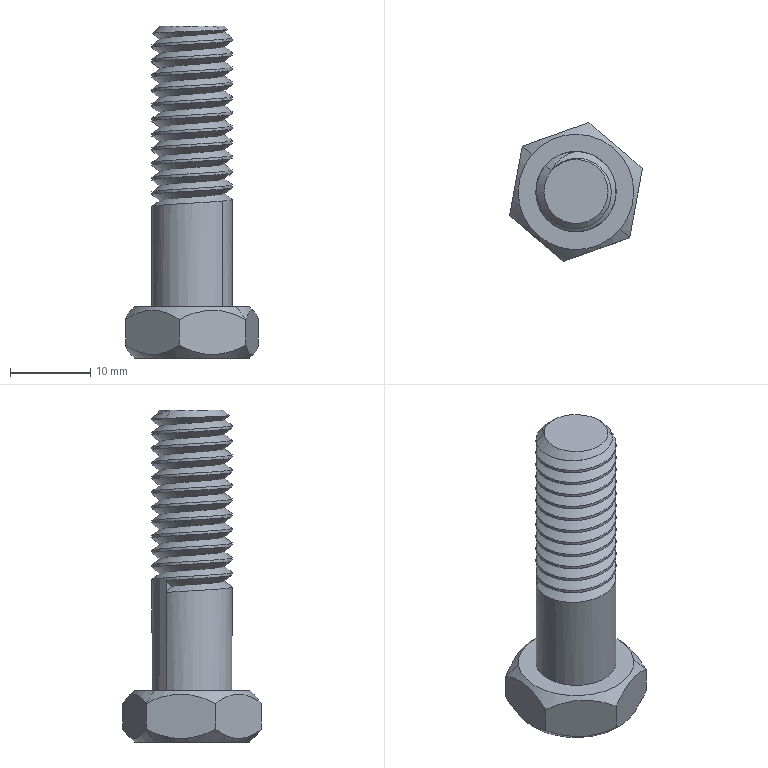Component | SolidWorks | M10-40-1 | 1 solid | 44 faces | volume 3726 mm3 | cylinder 25 | plane 10 | cone 7 | spline 2 | commonest cylinder face diameters 10 x25